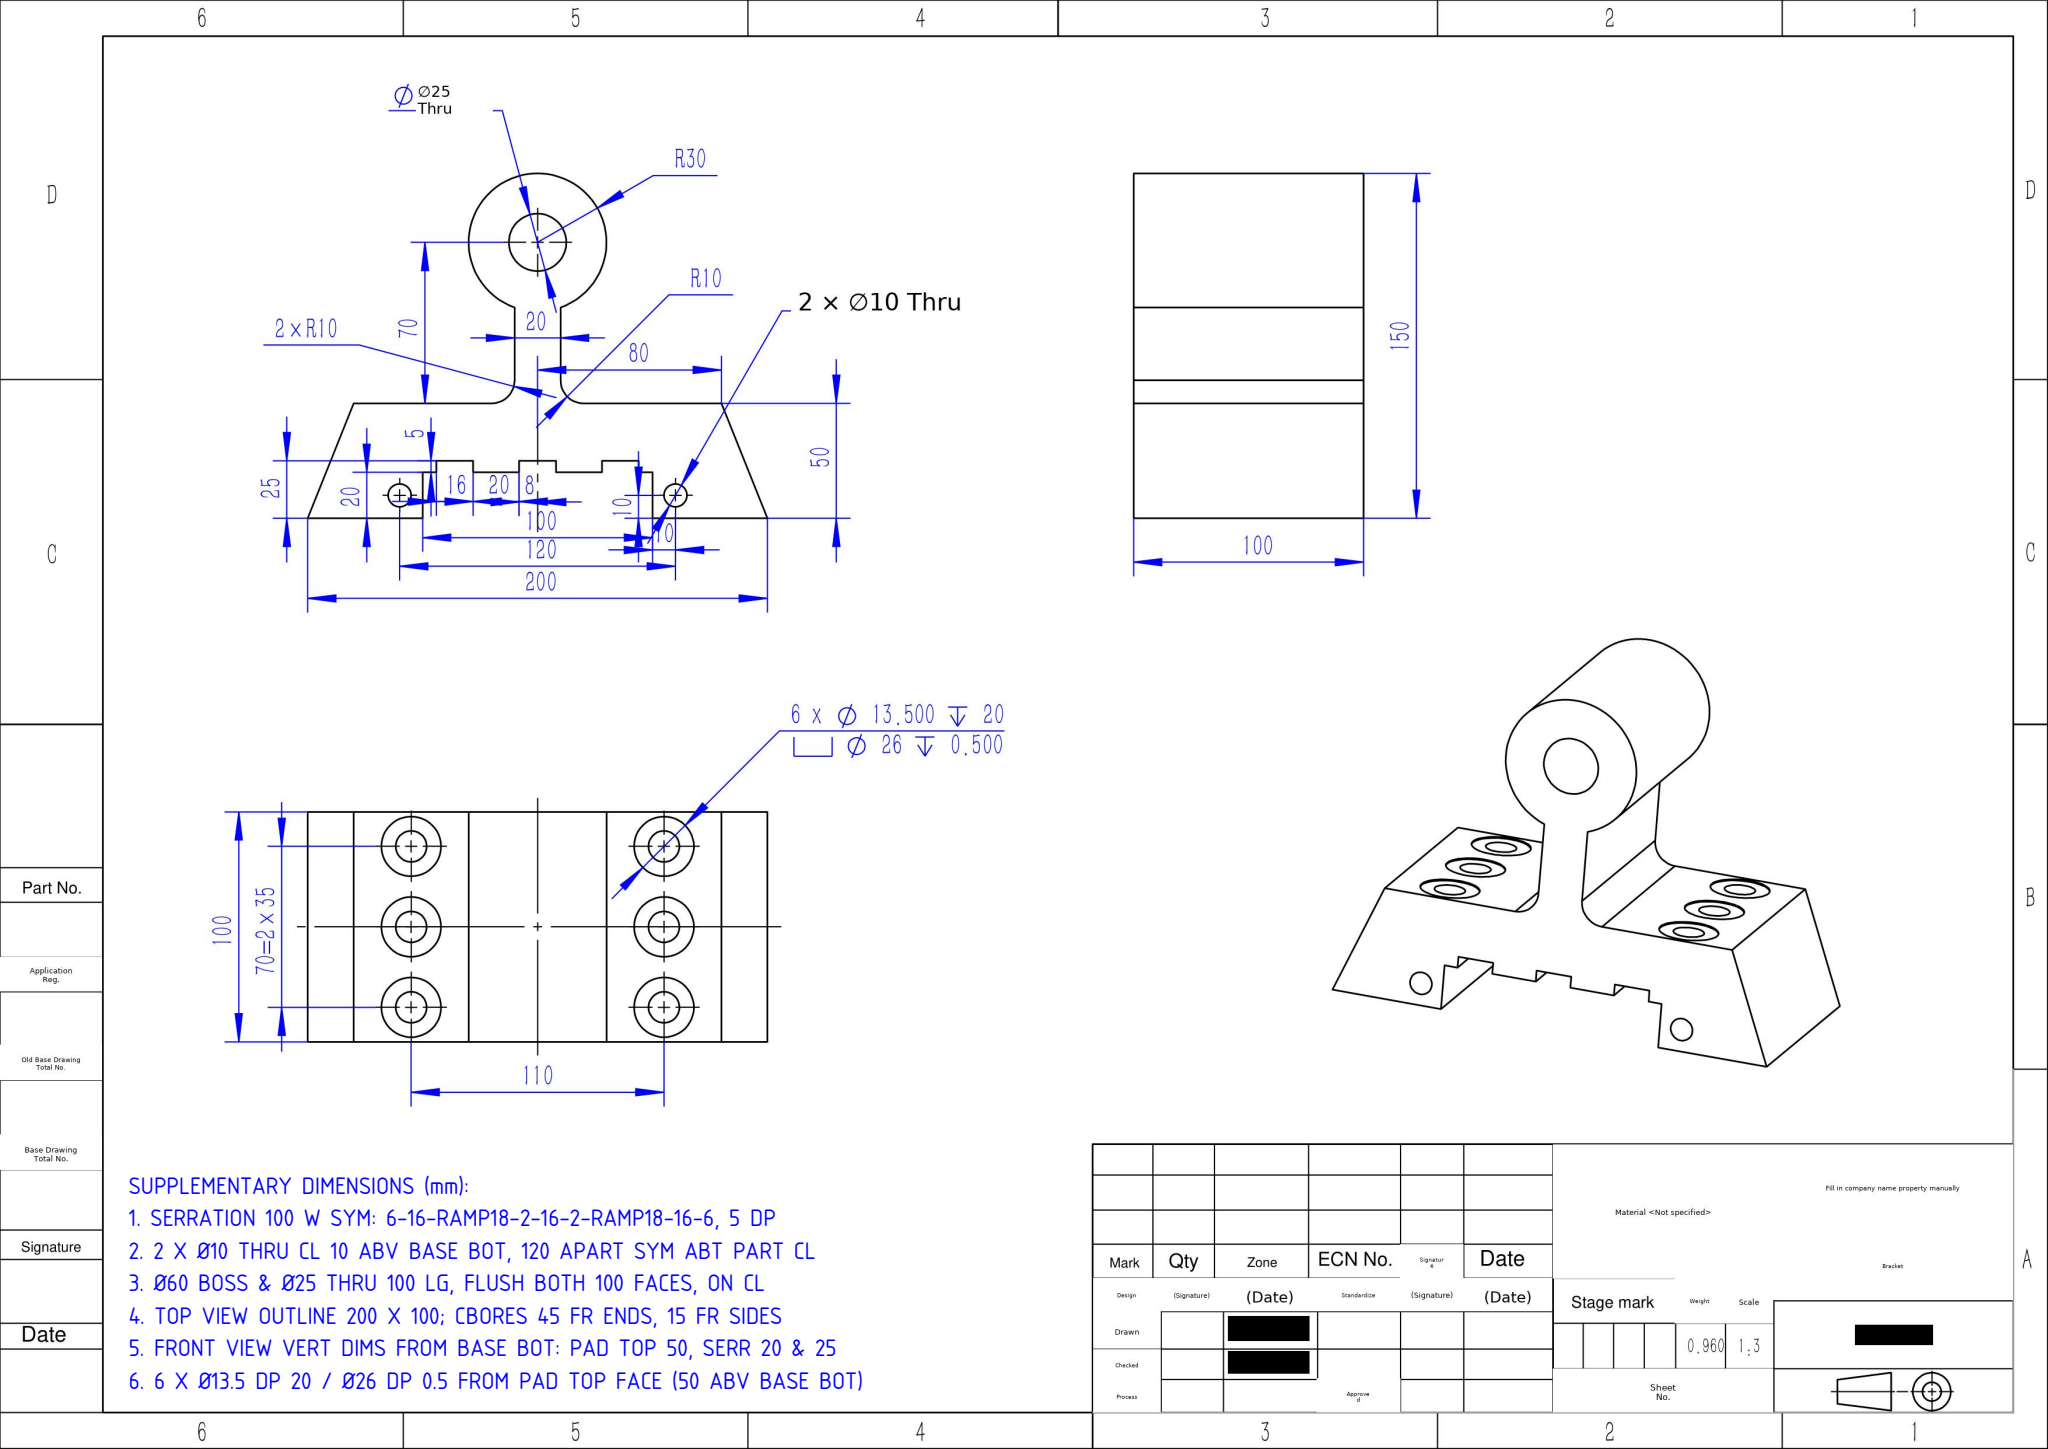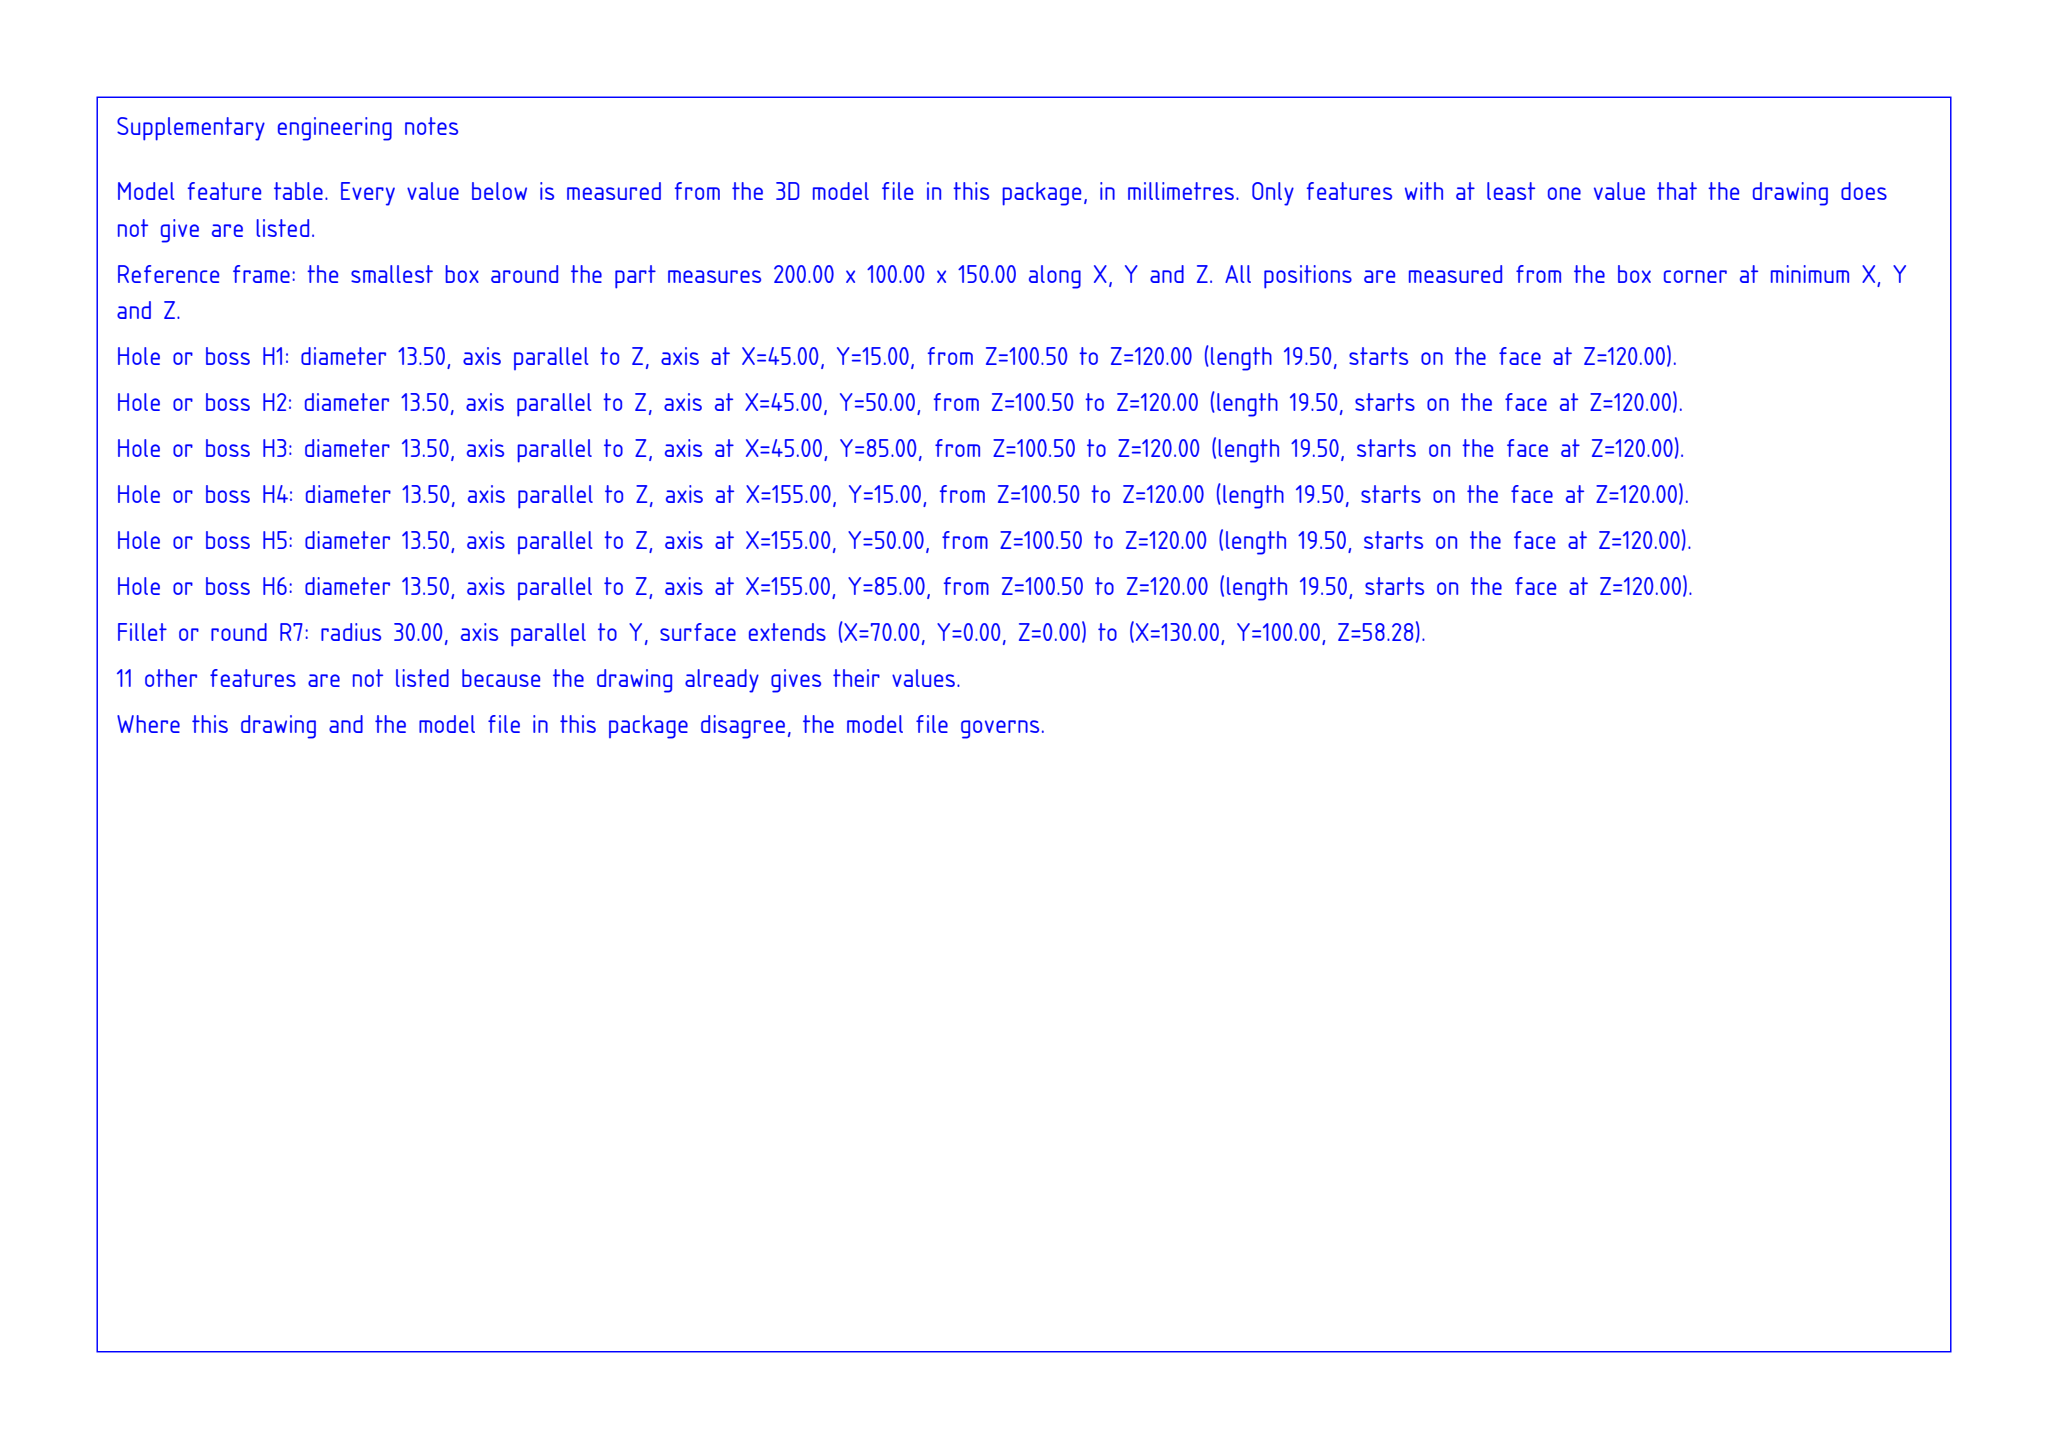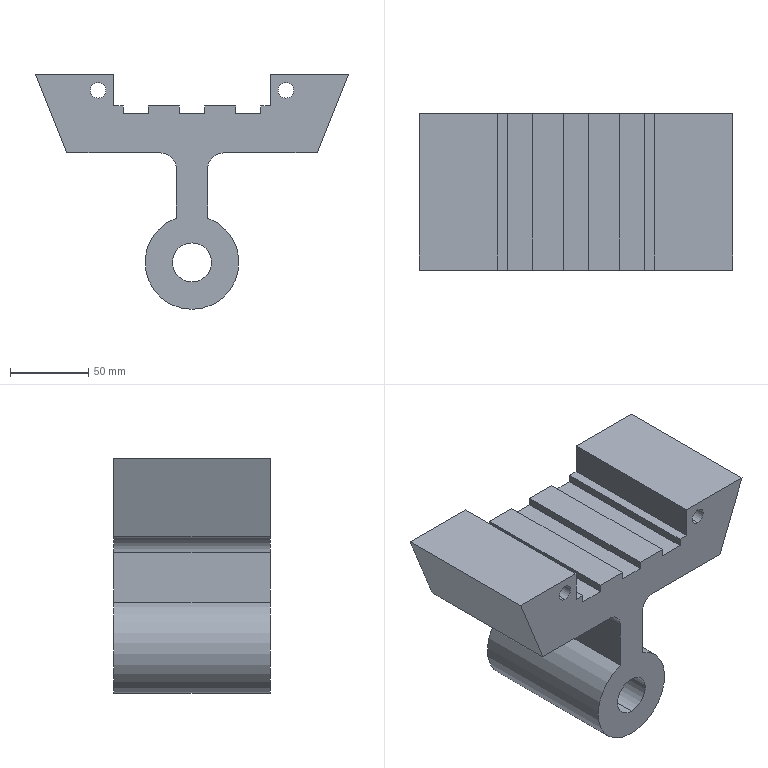Part | SolidWorks | mm | 1 solid | 77 faces | box 200 x 100 x 150 mm | volume 959869 mm3 | cylinder 34 | plane 31 | cone 12 | commonest cylinder face diameters 26 x12 13.5 x12 10 x4 25 x2 60 x2 20 x2
build123d program:
from build123d import *

# Parameters (mm, degrees)
BOSS_EXTRUDE1_DEPTH                                  = 50
BOSS_EXTRUDE2_DEPTH                                  = 50
SKETCH3_R                                            = 12.5
CUT_EXTRUDE1_DEPTH                                   = 207.155
FILLET1_R                                            = 10
SKETCH4_R                                            = 5
CUT_EXTRUDE2_DEPTH                                   = 207.155
CYLINDRICAL_COUNTERSUNK_HOLE_FOR_M12_HEX_D           = 13.5
CYLINDRICAL_COUNTERSUNK_HOLE_FOR_M12_HEX_DEPTH       = 20
CYLINDRICAL_COUNTERSUNK_HOLE_FOR_M12_HEX_CBORE_D     = 26
CYLINDRICAL_COUNTERSUNK_HOLE_FOR_M12_HEX_CBORE_DEPTH = 0.5
CYLINDRICAL_COUNTERSUNK_HOLE_FOR_M12_HEX_TIP         = 4.056
SKETCH8_W                                            = 16
SKETCH8_H                                            = 5
CUT_EXTRUDE3_DEPTH                                   = 207.155


with BuildPart() as part:
    # Sketch1 → Boss-Extrude1 (new, symmetric)
    with BuildSketch(Plane(origin=(0, 0, 0), x_dir=(1, 0, 0), z_dir=(0, 1, 0))):
        Polygon((100, 0), (50, 0), (50, 20), (-50, 20), (-50, 0), (-100, 0), (-80, 50), (80, 50), align=None)
    extrude(amount=BOSS_EXTRUDE1_DEPTH, both=True)

    # Sketch2 → Boss-Extrude2 (add, symmetric)
    with BuildSketch(Plane(origin=(0, 0, 0), x_dir=(1, 0, 0), z_dir=(0, 1, 0))):
        with BuildLine():
            Line((10, 50), (-10, 50))
            Line((-10, 50), (-10, 91.716))
            ThreePointArc((-10, 91.716), (0, 150), (10, 91.716))
            Line((10, 91.716), (10, 50))
        make_face()
    extrude(amount=BOSS_EXTRUDE2_DEPTH, both=True)

    # Sketch3 → Cut-Extrude1 (cut, through all)
    with BuildSketch(Plane.XZ.offset(50)):
        with Locations(Location((0, -120, 0), (0, 0, 270))):
            Circle(SKETCH3_R)
    extrude(amount=-CUT_EXTRUDE1_DEPTH, mode=Mode.SUBTRACT)

    # Fillet1
    fillet1_edges = [part.edges().sort_by_distance(p)[0] for p in [
        (10, 0, -50),
        (-10, 0, -50),
    ]]
    fillet(fillet1_edges, radius=FILLET1_R)

    # Sketch4 → Cut-Extrude2 (cut, through all)
    with BuildSketch(Plane.XZ.offset(50)):
        with Locations(Location((-60, -10, 0), (0, 0, 270))):
            Circle(SKETCH4_R)
        with Locations(Location((60, -10, 0), (0, 0, 90))):
            Circle(SKETCH4_R)
    extrude(amount=-CUT_EXTRUDE2_DEPTH, mode=Mode.SUBTRACT)

    # Cylindrical Countersunk Hole for M12 Hex
    with Locations(Plane(origin=(0, 0, -50), x_dir=(-1, 0, 0), z_dir=(0, 0, -1))):
        with Locations((-55, 35), (-55, 0), (-55, -35), (55, -35), (55, 0), (55, 35)):
            CounterBoreHole(CYLINDRICAL_COUNTERSUNK_HOLE_FOR_M12_HEX_D / 2, CYLINDRICAL_COUNTERSUNK_HOLE_FOR_M12_HEX_CBORE_D / 2, CYLINDRICAL_COUNTERSUNK_HOLE_FOR_M12_HEX_CBORE_DEPTH, depth=CYLINDRICAL_COUNTERSUNK_HOLE_FOR_M12_HEX_DEPTH)
            with Locations((0, 0, -(CYLINDRICAL_COUNTERSUNK_HOLE_FOR_M12_HEX_DEPTH + CYLINDRICAL_COUNTERSUNK_HOLE_FOR_M12_HEX_TIP / 2))):  # 118° drill point
                Cone(0, CYLINDRICAL_COUNTERSUNK_HOLE_FOR_M12_HEX_D / 2, CYLINDRICAL_COUNTERSUNK_HOLE_FOR_M12_HEX_TIP, mode=Mode.SUBTRACT)

    # Sketch8 → Cut-Extrude3 (cut, through all)
    with BuildSketch(Plane.XZ.offset(50)):
        with Locations((0, -22.5)):
            Rectangle(SKETCH8_W, SKETCH8_H)
        with Locations((36, -22.5)):
            Rectangle(SKETCH8_W, SKETCH8_H)
        with Locations((-36, -22.5)):
            Rectangle(SKETCH8_W, SKETCH8_H)
    extrude(amount=-CUT_EXTRUDE3_DEPTH, mode=Mode.SUBTRACT)


solid = part.part